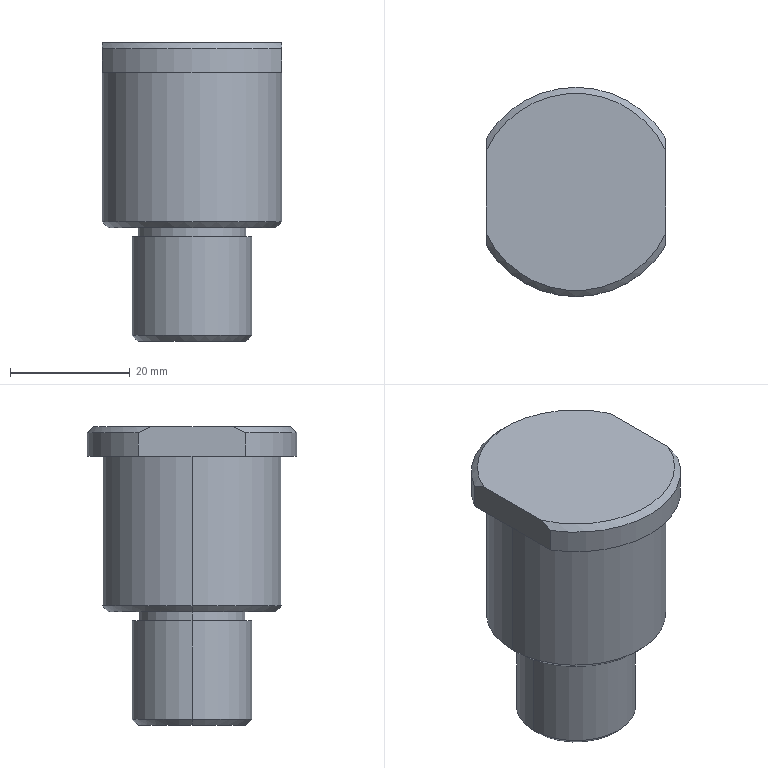Component | SolidWorks | M20Bolt1-1 | 1 solid | 22 faces | box 30 x 35 x 50 mm | volume 28650 mm3 | cylinder 8 | plane 8 | cone 6 | commonest cylinder face diameters 30 x2 18 x2 20 x2 35 x2
STEP:
#1=CARTESIAN_POINT('',(-3.691,40.171,0.315));
#2=VERTEX_POINT('',#1);
#3=CARTESIAN_POINT('',(-2.982,40.171,0.315));
#4=VERTEX_POINT('',#3);
#5=CARTESIAN_POINT('',(-3.336,40.171,0.315));
#6=DIRECTION('',(-0.,0.,-1.));
#7=DIRECTION('',(1.,0.,-0.));
#8=AXIS2_PLACEMENT_3D('',#5,#6,#7);
#9=CIRCLE('',#8,0.3543);
#10=EDGE_CURVE('',#2,#4,#9,.T.);
#11=ORIENTED_EDGE('',*,*,#10,.F.);
#12=CARTESIAN_POINT('',(-3.73,40.171,0.3543));
#13=VERTEX_POINT('',#12);
#14=CARTESIAN_POINT('',(-3.73,40.171,0.3543));
#15=DIRECTION('',(-0.7071,0.,0.7071));
#16=VECTOR('',#15,39.37);
#17=LINE('',#14,#16);
#18=EDGE_CURVE('',#2,#13,#17,.T.);
#19=ORIENTED_EDGE('',*,*,#18,.T.);
#20=CARTESIAN_POINT('',(-2.943,40.171,0.3543));
#21=VERTEX_POINT('',#20);
#22=CARTESIAN_POINT('',(-3.336,40.171,0.3543));
#23=DIRECTION('',(0.,0.,1.));
#24=DIRECTION('',(1.,0.,-0.));
#25=AXIS2_PLACEMENT_3D('',#22,#23,#24);
#26=CIRCLE('',#25,0.3937);
#27=EDGE_CURVE('',#21,#13,#26,.T.);
#28=ORIENTED_EDGE('',*,*,#27,.F.);
#29=CARTESIAN_POINT('',(-2.943,40.171,0.3543));
#30=DIRECTION('',(0.7071,0.,0.7071));
#31=VECTOR('',#30,39.37);
#32=LINE('',#29,#31);
#33=EDGE_CURVE('',#4,#21,#32,.T.);
#34=ORIENTED_EDGE('',*,*,#33,.F.);
#35=EDGE_LOOP('',(#11,#19,#28,#34));
#36=FACE_OUTER_BOUND('',#35,.T.);
#37=CARTESIAN_POINT('',(-3.336,40.171,0.3543));
#38=DIRECTION('',(0.,0.,1.));
#39=DIRECTION('',(1.,0.,-0.));
#40=AXIS2_PLACEMENT_3D('',#37,#38,#39);
#41=CONICAL_SURFACE('',#40,0.3937,0.7854);
#42=ADVANCED_FACE('',(#36),#41,.T.);
#43=CARTESIAN_POINT('',(-3.887,40.171,1.063));
#44=VERTEX_POINT('',#43);
#45=CARTESIAN_POINT('',(-2.785,40.171,1.063));
#46=VERTEX_POINT('',#45);
#47=CARTESIAN_POINT('',(-3.336,40.171,1.063));
#48=DIRECTION('',(-0.,0.,-1.));
#49=DIRECTION('',(1.,0.,-0.));
#50=AXIS2_PLACEMENT_3D('',#47,#48,#49);
#51=CIRCLE('',#50,0.5512);
#52=EDGE_CURVE('',#44,#46,#51,.T.);
#53=ORIENTED_EDGE('',*,*,#52,.F.);
#54=CARTESIAN_POINT('',(-3.927,40.171,1.102));
#55=VERTEX_POINT('',#54);
#56=CARTESIAN_POINT('',(-3.927,40.171,1.102));
#57=DIRECTION('',(-0.7071,0.,0.7071));
#58=VECTOR('',#57,39.37);
#59=LINE('',#56,#58);
#60=EDGE_CURVE('',#44,#55,#59,.T.);
#61=ORIENTED_EDGE('',*,*,#60,.T.);
#62=CARTESIAN_POINT('',(-2.746,40.171,1.102));
#63=VERTEX_POINT('',#62);
#64=CARTESIAN_POINT('',(-3.336,40.171,1.102));
#65=DIRECTION('',(0.,0.,1.));
#66=DIRECTION('',(1.,0.,-0.));
#67=AXIS2_PLACEMENT_3D('',#64,#65,#66);
#68=CIRCLE('',#67,0.5906);
#69=EDGE_CURVE('',#63,#55,#68,.T.);
#70=ORIENTED_EDGE('',*,*,#69,.F.);
#71=CARTESIAN_POINT('',(-2.746,40.171,1.102));
#72=DIRECTION('',(0.7071,0.,0.7071));
#73=VECTOR('',#72,39.37);
#74=LINE('',#71,#73);
#75=EDGE_CURVE('',#46,#63,#74,.T.);
#76=ORIENTED_EDGE('',*,*,#75,.F.);
#77=EDGE_LOOP('',(#53,#61,#70,#76));
#78=FACE_OUTER_BOUND('',#77,.T.);
#79=CARTESIAN_POINT('',(-3.336,40.171,1.102));
#80=DIRECTION('',(0.,0.,1.));
#81=DIRECTION('',(1.,0.,-0.));
#82=AXIS2_PLACEMENT_3D('',#79,#80,#81);
#83=CONICAL_SURFACE('',#82,0.5906,0.7854);
#84=ADVANCED_FACE('',(#78),#83,.T.);
#85=ORIENTED_EDGE('',*,*,#69,.T.);
#86=CARTESIAN_POINT('',(-3.927,40.171,2.087));
#87=VERTEX_POINT('',#86);
#88=CARTESIAN_POINT('',(-3.927,40.171,2.283));
#89=DIRECTION('',(0.,0.,1.));
#90=VECTOR('',#89,39.37);
#91=LINE('',#88,#90);
#92=EDGE_CURVE('',#55,#87,#91,.T.);
#93=ORIENTED_EDGE('',*,*,#92,.T.);
#94=CARTESIAN_POINT('',(-2.746,40.171,2.087));
#95=VERTEX_POINT('',#94);
#96=CARTESIAN_POINT('',(-3.336,40.171,2.087));
#97=DIRECTION('',(0.,0.,1.));
#98=DIRECTION('',(1.,0.,-0.));
#99=AXIS2_PLACEMENT_3D('',#96,#97,#98);
#100=CIRCLE('',#99,0.5906);
#101=EDGE_CURVE('',#95,#87,#100,.T.);
#102=ORIENTED_EDGE('',*,*,#101,.F.);
#103=CARTESIAN_POINT('',(-2.746,40.171,2.283));
#104=DIRECTION('',(0.,0.,1.));
#105=VECTOR('',#104,39.37);
#106=LINE('',#103,#105);
#107=EDGE_CURVE('',#63,#95,#106,.T.);
#108=ORIENTED_EDGE('',*,*,#107,.F.);
#109=EDGE_LOOP('',(#85,#93,#102,#108));
#110=FACE_OUTER_BOUND('',#109,.T.);
#111=CARTESIAN_POINT('',(-3.336,40.171,2.283));
#112=DIRECTION('',(0.,0.,1.));
#113=DIRECTION('',(1.,0.,-0.));
#114=AXIS2_PLACEMENT_3D('',#111,#112,#113);
#115=CYLINDRICAL_SURFACE('',#114,0.5906);
#116=ADVANCED_FACE('',(#110),#115,.T.);
#117=CARTESIAN_POINT('',(-2.982,40.171,1.004));
#118=VERTEX_POINT('',#117);
#119=CARTESIAN_POINT('',(-3.691,40.171,1.004));
#120=VERTEX_POINT('',#119);
#121=CARTESIAN_POINT('',(-3.336,40.171,1.004));
#122=DIRECTION('',(0.,0.,1.));
#123=DIRECTION('',(1.,0.,-0.));
#124=AXIS2_PLACEMENT_3D('',#121,#122,#123);
#125=CIRCLE('',#124,0.3543);
#126=EDGE_CURVE('',#118,#120,#125,.T.);
#127=ORIENTED_EDGE('',*,*,#126,.T.);
#128=CARTESIAN_POINT('',(-3.691,40.171,1.063));
#129=VERTEX_POINT('',#128);
#130=CARTESIAN_POINT('',(-3.691,40.171,2.283));
#131=DIRECTION('',(0.,0.,1.));
#132=VECTOR('',#131,39.37);
#133=LINE('',#130,#132);
#134=EDGE_CURVE('',#120,#129,#133,.T.);
#135=ORIENTED_EDGE('',*,*,#134,.T.);
#136=CARTESIAN_POINT('',(-2.982,40.171,1.063));
#137=VERTEX_POINT('',#136);
#138=CARTESIAN_POINT('',(-3.336,40.171,1.063));
#139=DIRECTION('',(0.,0.,1.));
#140=DIRECTION('',(1.,0.,-0.));
#141=AXIS2_PLACEMENT_3D('',#138,#139,#140);
#142=CIRCLE('',#141,0.3543);
#143=EDGE_CURVE('',#137,#129,#142,.T.);
#144=ORIENTED_EDGE('',*,*,#143,.F.);
#145=CARTESIAN_POINT('',(-2.982,40.171,2.283));
#146=DIRECTION('',(0.,0.,1.));
#147=VECTOR('',#146,39.37);
#148=LINE('',#145,#147);
#149=EDGE_CURVE('',#118,#137,#148,.T.);
#150=ORIENTED_EDGE('',*,*,#149,.F.);
#151=EDGE_LOOP('',(#127,#135,#144,#150));
#152=FACE_OUTER_BOUND('',#151,.T.);
#153=CARTESIAN_POINT('',(-3.336,40.171,2.283));
#154=DIRECTION('',(0.,0.,1.));
#155=DIRECTION('',(1.,0.,-0.));
#156=AXIS2_PLACEMENT_3D('',#153,#154,#155);
#157=CYLINDRICAL_SURFACE('',#156,0.3543);
#158=ADVANCED_FACE('',(#152),#157,.T.);
#159=ORIENTED_EDGE('',*,*,#27,.T.);
#160=CARTESIAN_POINT('',(-3.73,40.171,1.004));
#161=VERTEX_POINT('',#160);
#162=CARTESIAN_POINT('',(-3.73,40.171,2.283));
#163=DIRECTION('',(0.,0.,1.));
#164=VECTOR('',#163,39.37);
#165=LINE('',#162,#164);
#166=EDGE_CURVE('',#13,#161,#165,.T.);
#167=ORIENTED_EDGE('',*,*,#166,.T.);
#168=CARTESIAN_POINT('',(-2.943,40.171,1.004));
#169=VERTEX_POINT('',#168);
#170=CARTESIAN_POINT('',(-3.336,40.171,1.004));
#171=DIRECTION('',(0.,0.,1.));
#172=DIRECTION('',(1.,0.,-0.));
#173=AXIS2_PLACEMENT_3D('',#170,#171,#172);
#174=CIRCLE('',#173,0.3937);
#175=EDGE_CURVE('',#169,#161,#174,.T.);
#176=ORIENTED_EDGE('',*,*,#175,.F.);
#177=CARTESIAN_POINT('',(-2.943,40.171,2.283));
#178=DIRECTION('',(0.,0.,1.));
#179=VECTOR('',#178,39.37);
#180=LINE('',#177,#179);
#181=EDGE_CURVE('',#21,#169,#180,.T.);
#182=ORIENTED_EDGE('',*,*,#181,.F.);
#183=EDGE_LOOP('',(#159,#167,#176,#182));
#184=FACE_OUTER_BOUND('',#183,.T.);
#185=CARTESIAN_POINT('',(-3.336,40.171,2.283));
#186=DIRECTION('',(0.,0.,1.));
#187=DIRECTION('',(1.,0.,-0.));
#188=AXIS2_PLACEMENT_3D('',#185,#186,#187);
#189=CYLINDRICAL_SURFACE('',#188,0.3937);
#190=ADVANCED_FACE('',(#184),#189,.T.);
#191=CARTESIAN_POINT('',(-3.927,40.526,2.087));
#192=VERTEX_POINT('',#191);
#193=CARTESIAN_POINT('',(-3.927,38.971,2.087));
#194=DIRECTION('',(0.,-1.,0.));
#195=VECTOR('',#194,39.37);
#196=LINE('',#193,#195);
#197=EDGE_CURVE('',#192,#87,#196,.T.);
#198=ORIENTED_EDGE('',*,*,#197,.F.);
#199=CARTESIAN_POINT('',(-2.746,40.526,2.087));
#200=VERTEX_POINT('',#199);
#201=CARTESIAN_POINT('',(-3.336,40.171,2.087));
#202=DIRECTION('',(0.,0.,1.));
#203=DIRECTION('',(1.,0.,-0.));
#204=AXIS2_PLACEMENT_3D('',#201,#202,#203);
#205=CIRCLE('',#204,0.689);
#206=EDGE_CURVE('',#200,#192,#205,.T.);
#207=ORIENTED_EDGE('',*,*,#206,.F.);
#208=CARTESIAN_POINT('',(-2.746,38.971,2.087));
#209=DIRECTION('',(0.,1.,0.));
#210=VECTOR('',#209,39.37);
#211=LINE('',#208,#210);
#212=EDGE_CURVE('',#95,#200,#211,.T.);
#213=ORIENTED_EDGE('',*,*,#212,.F.);
#214=ORIENTED_EDGE('',*,*,#101,.T.);
#215=EDGE_LOOP('',(#198,#207,#213,#214));
#216=FACE_OUTER_BOUND('',#215,.T.);
#217=CARTESIAN_POINT('',(-3.336,40.762,2.087));
#218=DIRECTION('',(0.,0.,1.));
#219=DIRECTION('',(1.,0.,-0.));
#220=AXIS2_PLACEMENT_3D('',#217,#218,#219);
#221=PLANE('',#220);
#222=ADVANCED_FACE('',(#216),#221,.F.);
#223=CARTESIAN_POINT('',(-3.927,39.817,2.087));
#224=VERTEX_POINT('',#223);
#225=CARTESIAN_POINT('',(-3.927,38.971,2.087));
#226=DIRECTION('',(0.,-1.,0.));
#227=VECTOR('',#226,39.37);
#228=LINE('',#225,#227);
#229=EDGE_CURVE('',#87,#224,#228,.T.);
#230=ORIENTED_EDGE('',*,*,#229,.F.);
#231=CARTESIAN_POINT('',(-3.336,40.171,2.087));
#232=DIRECTION('',(0.,0.,1.));
#233=DIRECTION('',(1.,0.,-0.));
#234=AXIS2_PLACEMENT_3D('',#231,#232,#233);
#235=CIRCLE('',#234,0.5906);
#236=EDGE_CURVE('',#87,#95,#235,.T.);
#237=ORIENTED_EDGE('',*,*,#236,.T.);
#238=CARTESIAN_POINT('',(-2.746,39.817,2.087));
#239=VERTEX_POINT('',#238);
#240=CARTESIAN_POINT('',(-2.746,38.971,2.087));
#241=DIRECTION('',(0.,1.,0.));
#242=VECTOR('',#241,39.37);
#243=LINE('',#240,#242);
#244=EDGE_CURVE('',#239,#95,#243,.T.);
#245=ORIENTED_EDGE('',*,*,#244,.F.);
#246=CARTESIAN_POINT('',(-3.336,40.171,2.087));
#247=DIRECTION('',(0.,0.,1.));
#248=DIRECTION('',(1.,0.,-0.));
#249=AXIS2_PLACEMENT_3D('',#246,#247,#248);
#250=CIRCLE('',#249,0.689);
#251=EDGE_CURVE('',#224,#239,#250,.T.);
#252=ORIENTED_EDGE('',*,*,#251,.F.);
#253=EDGE_LOOP('',(#230,#237,#245,#252));
#254=FACE_OUTER_BOUND('',#253,.T.);
#255=CARTESIAN_POINT('',(-3.336,40.762,2.087));
#256=DIRECTION('',(0.,0.,1.));
#257=DIRECTION('',(1.,0.,-0.));
#258=AXIS2_PLACEMENT_3D('',#255,#256,#257);
#259=PLANE('',#258);
#260=ADVANCED_FACE('',(#254),#259,.F.);
#261=CARTESIAN_POINT('',(-3.927,39.817,2.244));
#262=VERTEX_POINT('',#261);
#263=CARTESIAN_POINT('',(-3.927,39.817,2.283));
#264=DIRECTION('',(0.,0.,1.));
#265=VECTOR('',#264,39.37);
#266=LINE('',#263,#265);
#267=EDGE_CURVE('',#224,#262,#266,.T.);
#268=ORIENTED_EDGE('',*,*,#267,.F.);
#269=ORIENTED_EDGE('',*,*,#251,.T.);
#270=CARTESIAN_POINT('',(-2.746,39.817,2.244));
#271=VERTEX_POINT('',#270);
#272=CARTESIAN_POINT('',(-2.746,39.817,2.283));
#273=DIRECTION('',(-0.,0.,-1.));
#274=VECTOR('',#273,39.37);
#275=LINE('',#272,#274);
#276=EDGE_CURVE('',#271,#239,#275,.T.);
#277=ORIENTED_EDGE('',*,*,#276,.F.);
#278=CARTESIAN_POINT('',(-3.336,40.171,2.244));
#279=DIRECTION('',(-0.,0.,-1.));
#280=DIRECTION('',(-1.,0.,0.));
#281=AXIS2_PLACEMENT_3D('',#278,#279,#280);
#282=CIRCLE('',#281,0.689);
#283=EDGE_CURVE('',#271,#262,#282,.T.);
#284=ORIENTED_EDGE('',*,*,#283,.T.);
#285=EDGE_LOOP('',(#268,#269,#277,#284));
#286=FACE_OUTER_BOUND('',#285,.T.);
#287=CARTESIAN_POINT('',(-3.336,40.171,2.283));
#288=DIRECTION('',(0.,0.,1.));
#289=DIRECTION('',(1.,0.,-0.));
#290=AXIS2_PLACEMENT_3D('',#287,#288,#289);
#291=CYLINDRICAL_SURFACE('',#290,0.689);
#292=ADVANCED_FACE('',(#286),#291,.T.);
#293=CARTESIAN_POINT('',(-3.927,40.526,2.244));
#294=VERTEX_POINT('',#293);
#295=CARTESIAN_POINT('',(-3.927,40.526,2.283));
#296=DIRECTION('',(-0.,0.,-1.));
#297=VECTOR('',#296,39.37);
#298=LINE('',#295,#297);
#299=EDGE_CURVE('',#294,#192,#298,.T.);
#300=ORIENTED_EDGE('',*,*,#299,.F.);
#301=CARTESIAN_POINT('',(-2.746,40.526,2.244));
#302=VERTEX_POINT('',#301);
#303=CARTESIAN_POINT('',(-3.336,40.171,2.244));
#304=DIRECTION('',(-0.,0.,-1.));
#305=DIRECTION('',(-1.,0.,0.));
#306=AXIS2_PLACEMENT_3D('',#303,#304,#305);
#307=CIRCLE('',#306,0.689);
#308=EDGE_CURVE('',#294,#302,#307,.T.);
#309=ORIENTED_EDGE('',*,*,#308,.T.);
#310=CARTESIAN_POINT('',(-2.746,40.526,2.283));
#311=DIRECTION('',(0.,0.,1.));
#312=VECTOR('',#311,39.37);
#313=LINE('',#310,#312);
#314=EDGE_CURVE('',#200,#302,#313,.T.);
#315=ORIENTED_EDGE('',*,*,#314,.F.);
#316=ORIENTED_EDGE('',*,*,#206,.T.);
#317=EDGE_LOOP('',(#300,#309,#315,#316));
#318=FACE_OUTER_BOUND('',#317,.T.);
#319=CARTESIAN_POINT('',(-3.336,40.171,2.283));
#320=DIRECTION('',(0.,0.,1.));
#321=DIRECTION('',(1.,0.,-0.));
#322=AXIS2_PLACEMENT_3D('',#319,#320,#321);
#323=CYLINDRICAL_SURFACE('',#322,0.689);
#324=ADVANCED_FACE('',(#318),#323,.T.);
#325=CARTESIAN_POINT('',(-3.927,40.442,2.283));
#326=VERTEX_POINT('',#325);
#327=CARTESIAN_POINT('',(-3.927,39.901,2.283));
#328=VERTEX_POINT('',#327);
#329=CARTESIAN_POINT('',(-3.927,38.971,2.283));
#330=DIRECTION('',(0.,-1.,0.));
#331=VECTOR('',#330,39.37);
#332=LINE('',#329,#331);
#333=EDGE_CURVE('',#326,#328,#332,.T.);
#334=ORIENTED_EDGE('',*,*,#333,.T.);
#335=CARTESIAN_POINT('',(-2.746,39.901,2.283));
#336=VERTEX_POINT('',#335);
#337=CARTESIAN_POINT('',(-3.336,40.171,2.283));
#338=DIRECTION('',(0.,0.,1.));
#339=DIRECTION('',(-1.,0.,0.));
#340=AXIS2_PLACEMENT_3D('',#337,#338,#339);
#341=CIRCLE('',#340,0.6496);
#342=EDGE_CURVE('',#328,#336,#341,.T.);
#343=ORIENTED_EDGE('',*,*,#342,.T.);
#344=CARTESIAN_POINT('',(-2.746,40.442,2.283));
#345=VERTEX_POINT('',#344);
#346=CARTESIAN_POINT('',(-2.746,38.971,2.283));
#347=DIRECTION('',(0.,1.,0.));
#348=VECTOR('',#347,39.37);
#349=LINE('',#346,#348);
#350=EDGE_CURVE('',#336,#345,#349,.T.);
#351=ORIENTED_EDGE('',*,*,#350,.T.);
#352=CARTESIAN_POINT('',(-3.336,40.171,2.283));
#353=DIRECTION('',(0.,0.,1.));
#354=DIRECTION('',(-1.,0.,0.));
#355=AXIS2_PLACEMENT_3D('',#352,#353,#354);
#356=CIRCLE('',#355,0.6496);
#357=EDGE_CURVE('',#345,#326,#356,.T.);
#358=ORIENTED_EDGE('',*,*,#357,.T.);
#359=EDGE_LOOP('',(#334,#343,#351,#358));
#360=FACE_OUTER_BOUND('',#359,.T.);
#361=CARTESIAN_POINT('',(-3.336,40.86,2.283));
#362=DIRECTION('',(-0.,0.,-1.));
#363=DIRECTION('',(-1.,0.,0.));
#364=AXIS2_PLACEMENT_3D('',#361,#362,#363);
#365=PLANE('',#364);
#366=ADVANCED_FACE('',(#360),#365,.F.);
#367=ORIENTED_EDGE('',*,*,#308,.F.);
#368=CARTESIAN_POINT('',(-3.927,40.526,2.244));
#369=CARTESIAN_POINT('',(-3.927,40.499,2.258));
#370=CARTESIAN_POINT('',(-3.927,40.471,2.272));
#371=CARTESIAN_POINT('',(-3.927,40.442,2.283));
#372=B_SPLINE_CURVE_WITH_KNOTS('',3,(#368,#369,#370,#371),.UNSPECIFIED.,.F.,.F.,(4,4),(0.03386,0.03623),.UNSPECIFIED.);
#373=EDGE_CURVE('',#294,#326,#372,.T.);
#374=ORIENTED_EDGE('',*,*,#373,.T.);
#375=ORIENTED_EDGE('',*,*,#357,.F.);
#376=CARTESIAN_POINT('',(-2.746,40.442,2.283));
#377=CARTESIAN_POINT('',(-2.746,40.471,2.271));
#378=CARTESIAN_POINT('',(-2.746,40.499,2.258));
#379=CARTESIAN_POINT('',(-2.746,40.526,2.244));
#380=B_SPLINE_CURVE_WITH_KNOTS('',3,(#376,#377,#378,#379),.UNSPECIFIED.,.F.,.F.,(4,4),(0.05039,0.05277),.UNSPECIFIED.);
#381=EDGE_CURVE('',#345,#302,#380,.T.);
#382=ORIENTED_EDGE('',*,*,#381,.T.);
#383=EDGE_LOOP('',(#367,#374,#375,#382));
#384=FACE_OUTER_BOUND('',#383,.T.);
#385=CARTESIAN_POINT('',(-3.336,40.171,2.283));
#386=DIRECTION('',(-0.,0.,-1.));
#387=DIRECTION('',(-1.,0.,0.));
#388=AXIS2_PLACEMENT_3D('',#385,#386,#387);
#389=CONICAL_SURFACE('',#388,0.6496,0.7854);
#390=ADVANCED_FACE('',(#384),#389,.T.);
#391=ORIENTED_EDGE('',*,*,#342,.F.);
#392=CARTESIAN_POINT('',(-3.927,39.901,2.283));
#393=CARTESIAN_POINT('',(-3.927,39.872,2.271));
#394=CARTESIAN_POINT('',(-3.927,39.844,2.258));
#395=CARTESIAN_POINT('',(-3.927,39.817,2.244));
#396=B_SPLINE_CURVE_WITH_KNOTS('',3,(#392,#393,#394,#395),.UNSPECIFIED.,.F.,.F.,(4,4),(0.05039,0.05277),.UNSPECIFIED.);
#397=EDGE_CURVE('',#328,#262,#396,.T.);
#398=ORIENTED_EDGE('',*,*,#397,.T.);
#399=ORIENTED_EDGE('',*,*,#283,.F.);
#400=CARTESIAN_POINT('',(-2.746,39.817,2.244));
#401=CARTESIAN_POINT('',(-2.746,39.844,2.258));
#402=CARTESIAN_POINT('',(-2.746,39.872,2.272));
#403=CARTESIAN_POINT('',(-2.746,39.901,2.283));
#404=B_SPLINE_CURVE_WITH_KNOTS('',3,(#400,#401,#402,#403),.UNSPECIFIED.,.F.,.F.,(4,4),(0.03386,0.03623),.UNSPECIFIED.);
#405=EDGE_CURVE('',#271,#336,#404,.T.);
#406=ORIENTED_EDGE('',*,*,#405,.T.);
#407=EDGE_LOOP('',(#391,#398,#399,#406));
#408=FACE_OUTER_BOUND('',#407,.T.);
#409=CARTESIAN_POINT('',(-3.336,40.171,2.283));
#410=DIRECTION('',(-0.,0.,-1.));
#411=DIRECTION('',(-1.,0.,0.));
#412=AXIS2_PLACEMENT_3D('',#409,#410,#411);
#413=CONICAL_SURFACE('',#412,0.6496,0.7854);
#414=ADVANCED_FACE('',(#408),#413,.T.);
#415=CARTESIAN_POINT('',(-3.336,40.171,0.315));
#416=DIRECTION('',(-0.,0.,-1.));
#417=DIRECTION('',(1.,0.,-0.));
#418=AXIS2_PLACEMENT_3D('',#415,#416,#417);
#419=CIRCLE('',#418,0.3543);
#420=EDGE_CURVE('',#4,#2,#419,.T.);
#421=ORIENTED_EDGE('',*,*,#420,.T.);
#422=ORIENTED_EDGE('',*,*,#10,.T.);
#423=EDGE_LOOP('',(#421,#422));
#424=FACE_OUTER_BOUND('',#423,.T.);
#425=CARTESIAN_POINT('',(-3.336,40.171,0.315));
#426=DIRECTION('',(0.,0.,1.));
#427=DIRECTION('',(1.,0.,-0.));
#428=AXIS2_PLACEMENT_3D('',#425,#426,#427);
#429=PLANE('',#428);
#430=ADVANCED_FACE('',(#424),#429,.F.);
#431=ORIENTED_EDGE('',*,*,#166,.F.);
#432=CARTESIAN_POINT('',(-3.336,40.171,0.3543));
#433=DIRECTION('',(0.,0.,1.));
#434=DIRECTION('',(1.,0.,-0.));
#435=AXIS2_PLACEMENT_3D('',#432,#433,#434);
#436=CIRCLE('',#435,0.3937);
#437=EDGE_CURVE('',#13,#21,#436,.T.);
#438=ORIENTED_EDGE('',*,*,#437,.T.);
#439=ORIENTED_EDGE('',*,*,#181,.T.);
#440=CARTESIAN_POINT('',(-3.336,40.171,1.004));
#441=DIRECTION('',(0.,0.,1.));
#442=DIRECTION('',(1.,0.,-0.));
#443=AXIS2_PLACEMENT_3D('',#440,#441,#442);
#444=CIRCLE('',#443,0.3937);
#445=EDGE_CURVE('',#161,#169,#444,.T.);
#446=ORIENTED_EDGE('',*,*,#445,.F.);
#447=EDGE_LOOP('',(#431,#438,#439,#446));
#448=FACE_OUTER_BOUND('',#447,.T.);
#449=CARTESIAN_POINT('',(-3.336,40.171,2.283));
#450=DIRECTION('',(0.,0.,1.));
#451=DIRECTION('',(1.,0.,-0.));
#452=AXIS2_PLACEMENT_3D('',#449,#450,#451);
#453=CYLINDRICAL_SURFACE('',#452,0.3937);
#454=ADVANCED_FACE('',(#448),#453,.T.);
#455=ORIENTED_EDGE('',*,*,#126,.F.);
#456=CARTESIAN_POINT('',(-3.336,40.171,1.004));
#457=DIRECTION('',(0.,0.,1.));
#458=DIRECTION('',(1.,0.,-0.));
#459=AXIS2_PLACEMENT_3D('',#456,#457,#458);
#460=CIRCLE('',#459,0.3543);
#461=EDGE_CURVE('',#120,#118,#460,.T.);
#462=ORIENTED_EDGE('',*,*,#461,.F.);
#463=EDGE_LOOP('',(#455,#462));
#464=FACE_BOUND('',#463,.T.);
#465=ORIENTED_EDGE('',*,*,#175,.T.);
#466=ORIENTED_EDGE('',*,*,#445,.T.);
#467=EDGE_LOOP('',(#465,#466));
#468=FACE_OUTER_BOUND('',#467,.T.);
#469=CARTESIAN_POINT('',(-3.336,40.565,1.004));
#470=DIRECTION('',(-0.,0.,-1.));
#471=DIRECTION('',(-1.,0.,0.));
#472=AXIS2_PLACEMENT_3D('',#469,#470,#471);
#473=PLANE('',#472);
#474=ADVANCED_FACE('',(#464,#468),#473,.F.);
#475=ORIENTED_EDGE('',*,*,#134,.F.);
#476=ORIENTED_EDGE('',*,*,#461,.T.);
#477=ORIENTED_EDGE('',*,*,#149,.T.);
#478=CARTESIAN_POINT('',(-3.336,40.171,1.063));
#479=DIRECTION('',(0.,0.,1.));
#480=DIRECTION('',(1.,0.,-0.));
#481=AXIS2_PLACEMENT_3D('',#478,#479,#480);
#482=CIRCLE('',#481,0.3543);
#483=EDGE_CURVE('',#129,#137,#482,.T.);
#484=ORIENTED_EDGE('',*,*,#483,.F.);
#485=EDGE_LOOP('',(#475,#476,#477,#484));
#486=FACE_OUTER_BOUND('',#485,.T.);
#487=CARTESIAN_POINT('',(-3.336,40.171,2.283));
#488=DIRECTION('',(0.,0.,1.));
#489=DIRECTION('',(1.,0.,-0.));
#490=AXIS2_PLACEMENT_3D('',#487,#488,#489);
#491=CYLINDRICAL_SURFACE('',#490,0.3543);
#492=ADVANCED_FACE('',(#486),#491,.T.);
#493=CARTESIAN_POINT('',(-3.336,40.171,1.063));
#494=DIRECTION('',(-0.,0.,-1.));
#495=DIRECTION('',(1.,0.,-0.));
#496=AXIS2_PLACEMENT_3D('',#493,#494,#495);
#497=CIRCLE('',#496,0.5512);
#498=EDGE_CURVE('',#46,#44,#497,.T.);
#499=ORIENTED_EDGE('',*,*,#498,.T.);
#500=ORIENTED_EDGE('',*,*,#52,.T.);
#501=EDGE_LOOP('',(#499,#500));
#502=FACE_OUTER_BOUND('',#501,.T.);
#503=ORIENTED_EDGE('',*,*,#143,.T.);
#504=ORIENTED_EDGE('',*,*,#483,.T.);
#505=EDGE_LOOP('',(#503,#504));
#506=FACE_BOUND('',#505,.T.);
#507=CARTESIAN_POINT('',(-3.336,40.526,1.063));
#508=DIRECTION('',(0.,0.,1.));
#509=DIRECTION('',(1.,0.,-0.));
#510=AXIS2_PLACEMENT_3D('',#507,#508,#509);
#511=PLANE('',#510);
#512=ADVANCED_FACE('',(#502,#506),#511,.F.);
#513=ORIENTED_EDGE('',*,*,#92,.F.);
#514=CARTESIAN_POINT('',(-3.336,40.171,1.102));
#515=DIRECTION('',(0.,0.,1.));
#516=DIRECTION('',(1.,0.,-0.));
#517=AXIS2_PLACEMENT_3D('',#514,#515,#516);
#518=CIRCLE('',#517,0.5906);
#519=EDGE_CURVE('',#55,#63,#518,.T.);
#520=ORIENTED_EDGE('',*,*,#519,.T.);
#521=ORIENTED_EDGE('',*,*,#107,.T.);
#522=ORIENTED_EDGE('',*,*,#236,.F.);
#523=EDGE_LOOP('',(#513,#520,#521,#522));
#524=FACE_OUTER_BOUND('',#523,.T.);
#525=CARTESIAN_POINT('',(-3.336,40.171,2.283));
#526=DIRECTION('',(0.,0.,1.));
#527=DIRECTION('',(1.,0.,-0.));
#528=AXIS2_PLACEMENT_3D('',#525,#526,#527);
#529=CYLINDRICAL_SURFACE('',#528,0.5906);
#530=ADVANCED_FACE('',(#524),#529,.T.);
#531=ORIENTED_EDGE('',*,*,#60,.F.);
#532=ORIENTED_EDGE('',*,*,#498,.F.);
#533=ORIENTED_EDGE('',*,*,#75,.T.);
#534=ORIENTED_EDGE('',*,*,#519,.F.);
#535=EDGE_LOOP('',(#531,#532,#533,#534));
#536=FACE_OUTER_BOUND('',#535,.T.);
#537=CARTESIAN_POINT('',(-3.336,40.171,1.102));
#538=DIRECTION('',(0.,0.,1.));
#539=DIRECTION('',(1.,0.,-0.));
#540=AXIS2_PLACEMENT_3D('',#537,#538,#539);
#541=CONICAL_SURFACE('',#540,0.5906,0.7854);
#542=ADVANCED_FACE('',(#536),#541,.T.);
#543=ORIENTED_EDGE('',*,*,#18,.F.);
#544=ORIENTED_EDGE('',*,*,#420,.F.);
#545=ORIENTED_EDGE('',*,*,#33,.T.);
#546=ORIENTED_EDGE('',*,*,#437,.F.);
#547=EDGE_LOOP('',(#543,#544,#545,#546));
#548=FACE_OUTER_BOUND('',#547,.T.);
#549=CARTESIAN_POINT('',(-3.336,40.171,0.3543));
#550=DIRECTION('',(0.,0.,1.));
#551=DIRECTION('',(1.,0.,-0.));
#552=AXIS2_PLACEMENT_3D('',#549,#550,#551);
#553=CONICAL_SURFACE('',#552,0.3937,0.7854);
#554=ADVANCED_FACE('',(#548),#553,.T.);
#555=ORIENTED_EDGE('',*,*,#276,.T.);
#556=ORIENTED_EDGE('',*,*,#244,.T.);
#557=ORIENTED_EDGE('',*,*,#212,.T.);
#558=ORIENTED_EDGE('',*,*,#314,.T.);
#559=ORIENTED_EDGE('',*,*,#381,.F.);
#560=ORIENTED_EDGE('',*,*,#350,.F.);
#561=ORIENTED_EDGE('',*,*,#405,.F.);
#562=EDGE_LOOP('',(#555,#556,#557,#558,#559,#560,#561));
#563=FACE_OUTER_BOUND('',#562,.T.);
#564=CARTESIAN_POINT('',(-2.746,38.971,2.087));
#565=DIRECTION('',(1.,0.,-0.));
#566=DIRECTION('',(-0.,0.,-1.));
#567=AXIS2_PLACEMENT_3D('',#564,#565,#566);
#568=PLANE('',#567);
#569=ADVANCED_FACE('',(#563),#568,.T.);
#570=ORIENTED_EDGE('',*,*,#299,.T.);
#571=ORIENTED_EDGE('',*,*,#197,.T.);
#572=ORIENTED_EDGE('',*,*,#229,.T.);
#573=ORIENTED_EDGE('',*,*,#267,.T.);
#574=ORIENTED_EDGE('',*,*,#397,.F.);
#575=ORIENTED_EDGE('',*,*,#333,.F.);
#576=ORIENTED_EDGE('',*,*,#373,.F.);
#577=EDGE_LOOP('',(#570,#571,#572,#573,#574,#575,#576));
#578=FACE_OUTER_BOUND('',#577,.T.);
#579=CARTESIAN_POINT('',(-3.927,38.971,2.087));
#580=DIRECTION('',(-1.,0.,0.));
#581=DIRECTION('',(0.,0.,1.));
#582=AXIS2_PLACEMENT_3D('',#579,#580,#581);
#583=PLANE('',#582);
#584=ADVANCED_FACE('',(#578),#583,.T.);
#585=CLOSED_SHELL('',(#42,#84,#116,#158,#190,#222,#260,#292,#324,#366,#390,#414,#430,#454,#474,#492,#512,#530,#542,#554,#569,#584));
#586=MANIFOLD_SOLID_BREP('',#585);
#587=CARTESIAN_POINT('',(0.,0.,0.));
#588=DIRECTION('',(0.,0.,1.));
#589=DIRECTION('',(1.,0.,0.));
#590=AXIS2_PLACEMENT_3D('',#587,#588,#589);
#591=(LENGTH_UNIT()NAMED_UNIT(*)SI_UNIT($,.METRE.));
#592=LENGTH_MEASURE_WITH_UNIT(LENGTH_MEASURE(0.0254),#591);
#593=DIMENSIONAL_EXPONENTS(1.,0.,0.,0.,0.,0.,0.);
#594=(CONVERSION_BASED_UNIT('',#592)LENGTH_UNIT()NAMED_UNIT(#593));
#595=UNCERTAINTY_MEASURE_WITH_UNIT(LENGTH_MEASURE(0.00001),#594,'','');
#596=(NAMED_UNIT(*)PLANE_ANGLE_UNIT()SI_UNIT($,.RADIAN.));
#597=(NAMED_UNIT(*)SI_UNIT($,.STERADIAN.)SOLID_ANGLE_UNIT());
#598=(GEOMETRIC_REPRESENTATION_CONTEXT(3)GLOBAL_UNCERTAINTY_ASSIGNED_CONTEXT((#595))GLOBAL_UNIT_ASSIGNED_CONTEXT((#594,#596,#597))REPRESENTATION_CONTEXT('',''));
#599=ADVANCED_BREP_SHAPE_REPRESENTATION('',(#586,#590),#598);
#600=COLOUR_RGB('',0.7922,0.8196,0.9333);
#601=FILL_AREA_STYLE_COLOUR('',#600);
#602=FILL_AREA_STYLE('',(#601));
#603=SURFACE_STYLE_FILL_AREA(#602);
#604=SURFACE_SIDE_STYLE('',(#603));
#605=SURFACE_STYLE_USAGE(.BOTH.,#604);
#606=PRESENTATION_STYLE_ASSIGNMENT((#605));
#607=STYLED_ITEM('',(#606),#586);
#608=PRESENTATION_LAYER_ASSIGNMENT('','',(#607));
#609=(LENGTH_UNIT()NAMED_UNIT(*)SI_UNIT($,.METRE.));
#610=LENGTH_MEASURE_WITH_UNIT(LENGTH_MEASURE(0.0254),#609);
#611=DIMENSIONAL_EXPONENTS(1.,0.,0.,0.,0.,0.,0.);
#612=(CONVERSION_BASED_UNIT('',#610)LENGTH_UNIT()NAMED_UNIT(#611));
#613=UNCERTAINTY_MEASURE_WITH_UNIT(LENGTH_MEASURE(0.00001),#612,'','');
#614=(NAMED_UNIT(*)PLANE_ANGLE_UNIT()SI_UNIT($,.RADIAN.));
#615=(NAMED_UNIT(*)SI_UNIT($,.STERADIAN.)SOLID_ANGLE_UNIT());
#616=(GEOMETRIC_REPRESENTATION_CONTEXT(3)GLOBAL_UNCERTAINTY_ASSIGNED_CONTEXT((#613))GLOBAL_UNIT_ASSIGNED_CONTEXT((#612,#614,#615))REPRESENTATION_CONTEXT('',''));
#617=MECHANICAL_DESIGN_GEOMETRIC_PRESENTATION_REPRESENTATION('',(#607),#616);